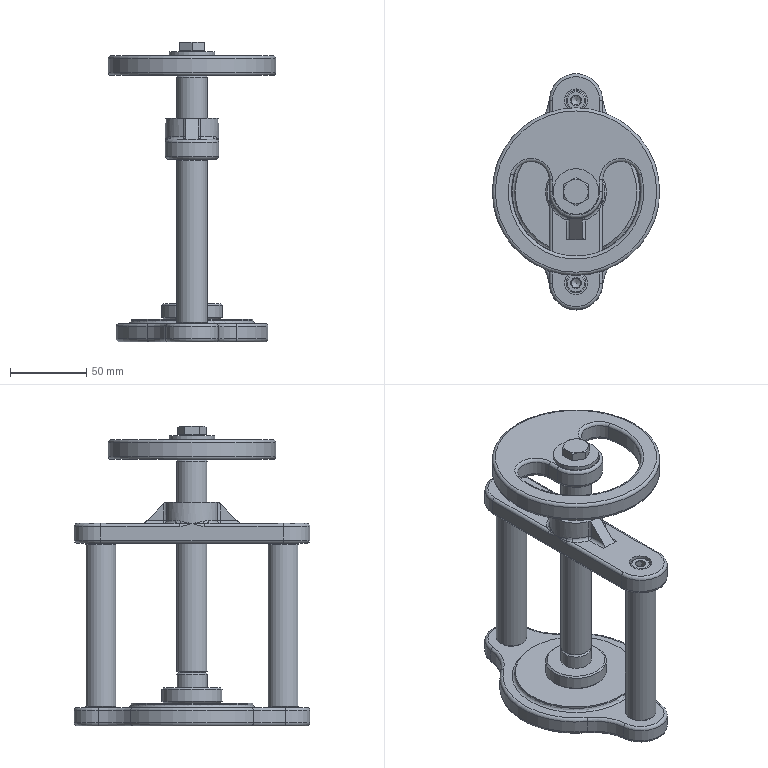Assembly | NX | mm | 13 component files | 13 solids | 296 faces | box 110 x 155 x 196.9 mm | volume 408324 mm3 | plane 106 | cylinder 72 | cone 58 | torus 44 | spline 12 | sphere 4 | commonest cylinder face diameters 4 x18 35 x7 20 x5 9 x5 15 x5 8 x4 7.76 x4 13 x4
Bill of materials:
unnamed part 1 | 2 |  | Long, slender straight cylinder with a small central axial bore, like a tube or spacer, with small chamfers at both ends.
unnamed part 2 | 1 |  | Stepped round bushing: a wide, short disc flange with a smaller cylindrical boss on one side and a central through-hole, chamfered on its outer edges.
unnamed part 3 | 1 |  | Thin round disc with rounded edges. A large curved cutout leaves an outer ring joined to a central tongue, and the tongue has a small round hole.
GB-T96_1-2002,M10 | 1 |  | Thin, flat annular disc (plain washer-like ring) with a single concentric circular through-hole and parallel flat faces.
unnamed part 4 | 1 |  | Flat bar with rounded ends and a small hole near each end. At the centre is a raised cylindrical boss with a larger through-hole, braced by two triangular ribs along the bar's long axis.
unnamed part 5 | 1 |  | Long, slender hollow cylinder with a short, smaller-diameter stepped section at one end and an axial bore.
GB-T5782-2000,M10x20 | 1 |  | Hexagon Head Bolt, GB-T 5782-2000,M10x20
GB-T70.1-2000,M8x16 | 4 |  | Hexagon Socket Head Cap Screw, GB-T 70.1-2000,M8x16
unnamed part 6 | 1 |  | Flat plate with two lobes: a central round body and two rounded ear tabs on opposite sides, each tab with a small hole. A shallow, slightly raised circular face sits on top of the central body.
Mates:
1. fix | base 1 component
2. concentric | GB-T96_1-2002_M10 1 edge | handle 1 edge
3. concentric | GB-T5782-2000_M10x20 1 edge | GB-T96_1-2002_M10 1 edge